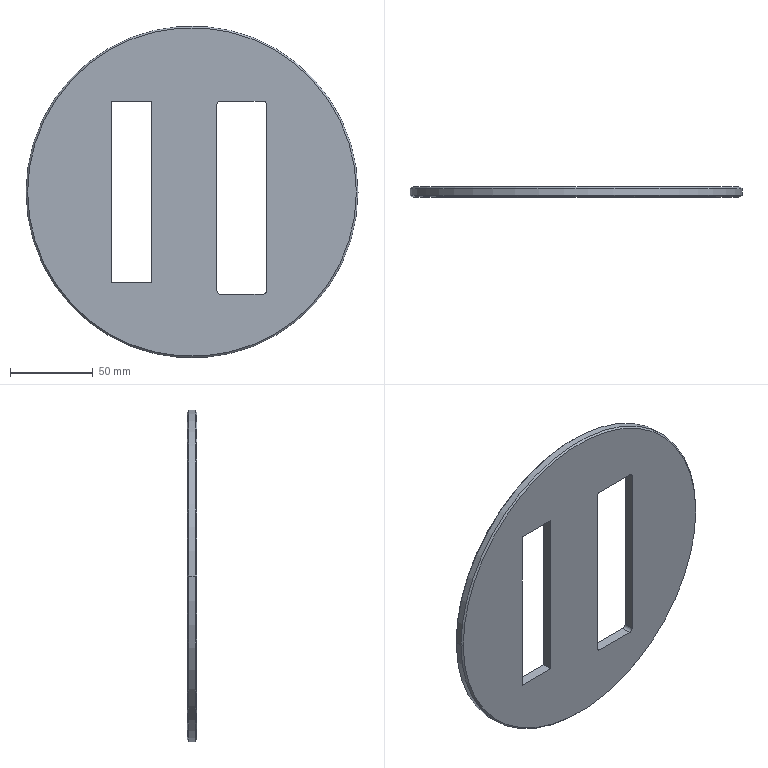Component | SolidWorks | Inline-H010-H01160308-003K-1 | 1 solid | 20 faces | box 200 x 6 x 200 mm | volume 151116 mm3 | plane 10 | cylinder 6 | cone 4 | commonest cylinder face diameters 4 x4 200 x2
build123d program:
from build123d import *

# Parameters (mm, degrees)
SKETCH1_R           = 100
BOSS_EXTRUDE1_DEPTH = 3
CHAMFER1_SIZE       = 1
SKETCH2_W           = 24.288
SKETCH2_H           = 109.389
CUT_EXTRUDE1_DEPTH  = 10


with BuildPart() as part:
    # Sketch1 → Boss-Extrude1 (new, symmetric)
    with BuildSketch(Plane.XY):
        Circle(SKETCH1_R)
    extrude(amount=BOSS_EXTRUDE1_DEPTH, both=True)

    # Chamfer1
    chamfer1_edges = [part.edges().sort_by_distance(p)[0] for p in [
        (-100, 0, -3),
        (-100, 0, 3),
    ]]
    chamfer(chamfer1_edges, length=CHAMFER1_SIZE)

    # Sketch2 → Cut-Extrude1 (cut)
    with BuildSketch(Plane(origin=(0, 0, -3), x_dir=(-1, 0, 0), z_dir=(0, 0, -1))):
        with BuildLine():
            Line((-17.028, -61.574), (-42.891, -61.574))
            ThreePointArc((-42.891, -61.574), (-44.305, -60.989), (-44.891, -59.574))
            Line((-44.891, -59.574), (-44.891, 52.695))
            ThreePointArc((-44.891, 52.695), (-44.305, 54.109), (-42.891, 54.695))
            Line((-42.891, 54.695), (-17.028, 54.695))
            ThreePointArc((-17.028, 54.695), (-15.614, 54.109), (-15.028, 52.695))
            Line((-15.028, 52.695), (-15.028, -59.574))
            ThreePointArc((-15.028, -59.574), (-15.614, -60.989), (-17.028, -61.574))
        make_face()
        with Locations((36.583, 0)):
            Rectangle(SKETCH2_W, SKETCH2_H)
    extrude(amount=-CUT_EXTRUDE1_DEPTH, mode=Mode.SUBTRACT)


solid = part.part

# Placed as in the assembly
solid = solid.moved(Location((29.082, 23.968, 139.665), (90, 0, 0)))
STEP:
#1=COLOUR_RGB('',0.7922,0.8196,0.9333);
#2=FILL_AREA_STYLE_COLOUR('',#1);
#3=FILL_AREA_STYLE('',(#2));
#4=SURFACE_STYLE_FILL_AREA(#3);
#5=SURFACE_SIDE_STYLE('',(#4));
#6=SURFACE_STYLE_USAGE(.BOTH.,#5);
#7=PRESENTATION_STYLE_ASSIGNMENT((#6));
#8=CARTESIAN_POINT('',(-2.753,1.062,5.499));
#9=VERTEX_POINT('',#8);
#10=CARTESIAN_POINT('',(5.043,1.062,5.499));
#11=VERTEX_POINT('',#10);
#12=CARTESIAN_POINT('',(1.145,1.062,5.499));
#13=DIRECTION('',(0.,1.,0.));
#14=DIRECTION('',(1.,-0.,0.));
#15=AXIS2_PLACEMENT_3D('',#12,#13,#14);
#16=CIRCLE('',#15,3.898);
#17=EDGE_CURVE('',#9,#11,#16,.T.);
#18=ORIENTED_EDGE('',*,*,#17,.F.);
#19=CARTESIAN_POINT('',(-2.792,1.022,5.499));
#20=VERTEX_POINT('',#19);
#21=CARTESIAN_POINT('',(-2.792,1.022,5.499));
#22=DIRECTION('',(-0.7071,-0.7071,0.));
#23=VECTOR('',#22,39.37);
#24=LINE('',#21,#23);
#25=EDGE_CURVE('',#9,#20,#24,.T.);
#26=ORIENTED_EDGE('',*,*,#25,.T.);
#27=CARTESIAN_POINT('',(5.082,1.022,5.499));
#28=VERTEX_POINT('',#27);
#29=CARTESIAN_POINT('',(1.145,1.022,5.499));
#30=DIRECTION('',(-0.,-1.,-0.));
#31=DIRECTION('',(1.,-0.,0.));
#32=AXIS2_PLACEMENT_3D('',#29,#30,#31);
#33=CIRCLE('',#32,3.937);
#34=EDGE_CURVE('',#28,#20,#33,.T.);
#35=ORIENTED_EDGE('',*,*,#34,.F.);
#36=CARTESIAN_POINT('',(5.082,1.022,5.499));
#37=DIRECTION('',(0.7071,-0.7071,-0.));
#38=VECTOR('',#37,39.37);
#39=LINE('',#36,#38);
#40=EDGE_CURVE('',#11,#28,#39,.T.);
#41=ORIENTED_EDGE('',*,*,#40,.F.);
#42=EDGE_LOOP('',(#18,#26,#35,#41));
#43=FACE_OUTER_BOUND('',#42,.T.);
#44=CARTESIAN_POINT('',(1.145,1.022,5.499));
#45=DIRECTION('',(-0.,-1.,-0.));
#46=DIRECTION('',(1.,-0.,0.));
#47=AXIS2_PLACEMENT_3D('',#44,#45,#46);
#48=CONICAL_SURFACE('',#47,3.937,0.7854);
#49=ADVANCED_FACE('',(#43),#48,.T.);
#50=CARTESIAN_POINT('',(5.043,0.8255,5.499));
#51=VERTEX_POINT('',#50);
#52=CARTESIAN_POINT('',(-2.753,0.8255,5.499));
#53=VERTEX_POINT('',#52);
#54=CARTESIAN_POINT('',(1.145,0.8255,5.499));
#55=DIRECTION('',(-0.,-1.,-0.));
#56=DIRECTION('',(1.,-0.,0.));
#57=AXIS2_PLACEMENT_3D('',#54,#55,#56);
#58=CIRCLE('',#57,3.898);
#59=EDGE_CURVE('',#51,#53,#58,.T.);
#60=ORIENTED_EDGE('',*,*,#59,.F.);
#61=CARTESIAN_POINT('',(5.082,0.8649,5.499));
#62=VERTEX_POINT('',#61);
#63=CARTESIAN_POINT('',(5.043,0.8255,5.499));
#64=DIRECTION('',(0.7071,0.7071,0.));
#65=VECTOR('',#64,39.37);
#66=LINE('',#63,#65);
#67=EDGE_CURVE('',#51,#62,#66,.T.);
#68=ORIENTED_EDGE('',*,*,#67,.T.);
#69=CARTESIAN_POINT('',(-2.792,0.8649,5.499));
#70=VERTEX_POINT('',#69);
#71=CARTESIAN_POINT('',(1.145,0.8649,5.499));
#72=DIRECTION('',(0.,1.,0.));
#73=DIRECTION('',(1.,-0.,0.));
#74=AXIS2_PLACEMENT_3D('',#71,#72,#73);
#75=CIRCLE('',#74,3.937);
#76=EDGE_CURVE('',#70,#62,#75,.T.);
#77=ORIENTED_EDGE('',*,*,#76,.F.);
#78=CARTESIAN_POINT('',(-2.753,0.8255,5.499));
#79=DIRECTION('',(-0.7071,0.7071,0.));
#80=VECTOR('',#79,39.37);
#81=LINE('',#78,#80);
#82=EDGE_CURVE('',#53,#70,#81,.T.);
#83=ORIENTED_EDGE('',*,*,#82,.F.);
#84=EDGE_LOOP('',(#60,#68,#77,#83));
#85=FACE_OUTER_BOUND('',#84,.T.);
#86=CARTESIAN_POINT('',(1.145,0.8255,5.499));
#87=DIRECTION('',(0.,1.,0.));
#88=DIRECTION('',(-1.,0.,0.));
#89=AXIS2_PLACEMENT_3D('',#86,#87,#88);
#90=CONICAL_SURFACE('',#89,3.898,0.7854);
#91=ADVANCED_FACE('',(#85),#90,.T.);
#92=ORIENTED_EDGE('',*,*,#76,.T.);
#93=CARTESIAN_POINT('',(5.082,0.8255,5.499));
#94=DIRECTION('',(0.,1.,0.));
#95=VECTOR('',#94,39.37);
#96=LINE('',#93,#95);
#97=EDGE_CURVE('',#62,#28,#96,.T.);
#98=ORIENTED_EDGE('',*,*,#97,.T.);
#99=ORIENTED_EDGE('',*,*,#34,.T.);
#100=CARTESIAN_POINT('',(-2.792,0.8255,5.499));
#101=DIRECTION('',(0.,1.,0.));
#102=VECTOR('',#101,39.37);
#103=LINE('',#100,#102);
#104=EDGE_CURVE('',#70,#20,#103,.T.);
#105=ORIENTED_EDGE('',*,*,#104,.F.);
#106=EDGE_LOOP('',(#92,#98,#99,#105));
#107=FACE_OUTER_BOUND('',#106,.T.);
#108=CARTESIAN_POINT('',(1.145,0.8255,5.499));
#109=DIRECTION('',(0.,1.,0.));
#110=DIRECTION('',(-1.,0.,0.));
#111=AXIS2_PLACEMENT_3D('',#108,#109,#110);
#112=CYLINDRICAL_SURFACE('',#111,3.937);
#113=ADVANCED_FACE('',(#107),#112,.T.);
#114=ORIENTED_EDGE('',*,*,#97,.F.);
#115=CARTESIAN_POINT('',(1.145,0.8649,5.499));
#116=DIRECTION('',(0.,1.,0.));
#117=DIRECTION('',(1.,-0.,0.));
#118=AXIS2_PLACEMENT_3D('',#115,#116,#117);
#119=CIRCLE('',#118,3.937);
#120=EDGE_CURVE('',#62,#70,#119,.T.);
#121=ORIENTED_EDGE('',*,*,#120,.T.);
#122=ORIENTED_EDGE('',*,*,#104,.T.);
#123=CARTESIAN_POINT('',(1.145,1.022,5.499));
#124=DIRECTION('',(-0.,-1.,-0.));
#125=DIRECTION('',(1.,-0.,0.));
#126=AXIS2_PLACEMENT_3D('',#123,#124,#125);
#127=CIRCLE('',#126,3.937);
#128=EDGE_CURVE('',#20,#28,#127,.T.);
#129=ORIENTED_EDGE('',*,*,#128,.T.);
#130=EDGE_LOOP('',(#114,#121,#122,#129));
#131=FACE_OUTER_BOUND('',#130,.T.);
#132=CARTESIAN_POINT('',(1.145,0.8255,5.499));
#133=DIRECTION('',(0.,1.,0.));
#134=DIRECTION('',(-1.,0.,0.));
#135=AXIS2_PLACEMENT_3D('',#132,#133,#134);
#136=CYLINDRICAL_SURFACE('',#135,3.937);
#137=ADVANCED_FACE('',(#131),#136,.T.);
#138=CARTESIAN_POINT('',(0.1828,0.8255,3.345));
#139=VERTEX_POINT('',#138);
#140=CARTESIAN_POINT('',(0.1828,0.8255,7.652));
#141=VERTEX_POINT('',#140);
#142=CARTESIAN_POINT('',(0.1828,0.8255,5.499));
#143=DIRECTION('',(0.,-0.,1.));
#144=VECTOR('',#143,39.37);
#145=LINE('',#142,#144);
#146=EDGE_CURVE('',#139,#141,#145,.T.);
#147=ORIENTED_EDGE('',*,*,#146,.F.);
#148=CARTESIAN_POINT('',(-0.7734,0.8255,3.345));
#149=VERTEX_POINT('',#148);
#150=CARTESIAN_POINT('',(1.145,0.8255,3.345));
#151=DIRECTION('',(1.,-0.,-0.));
#152=VECTOR('',#151,39.37);
#153=LINE('',#150,#152);
#154=EDGE_CURVE('',#149,#139,#153,.T.);
#155=ORIENTED_EDGE('',*,*,#154,.F.);
#156=CARTESIAN_POINT('',(-0.7734,0.8255,7.652));
#157=VERTEX_POINT('',#156);
#158=CARTESIAN_POINT('',(-0.7734,0.8255,5.499));
#159=DIRECTION('',(-0.,0.,-1.));
#160=VECTOR('',#159,39.37);
#161=LINE('',#158,#160);
#162=EDGE_CURVE('',#157,#149,#161,.T.);
#163=ORIENTED_EDGE('',*,*,#162,.F.);
#164=CARTESIAN_POINT('',(1.145,0.8255,7.652));
#165=DIRECTION('',(-1.,0.,0.));
#166=VECTOR('',#165,39.37);
#167=LINE('',#164,#166);
#168=EDGE_CURVE('',#141,#157,#167,.T.);
#169=ORIENTED_EDGE('',*,*,#168,.F.);
#170=EDGE_LOOP('',(#147,#155,#163,#169));
#171=FACE_BOUND('',#170,.T.);
#172=CARTESIAN_POINT('',(1.737,0.8255,3.153));
#173=VERTEX_POINT('',#172);
#174=CARTESIAN_POINT('',(1.815,0.8255,3.074));
#175=VERTEX_POINT('',#174);
#176=CARTESIAN_POINT('',(1.815,0.8255,3.153));
#177=DIRECTION('',(-0.,-1.,-0.));
#178=DIRECTION('',(1.,0.,0.));
#179=AXIS2_PLACEMENT_3D('',#176,#177,#178);
#180=CIRCLE('',#179,0.07874);
#181=EDGE_CURVE('',#173,#175,#180,.T.);
#182=ORIENTED_EDGE('',*,*,#181,.F.);
#183=CARTESIAN_POINT('',(1.737,0.8255,7.573));
#184=VERTEX_POINT('',#183);
#185=CARTESIAN_POINT('',(1.737,0.8255,5.499));
#186=DIRECTION('',(-0.,0.,-1.));
#187=VECTOR('',#186,39.37);
#188=LINE('',#185,#187);
#189=EDGE_CURVE('',#184,#173,#188,.T.);
#190=ORIENTED_EDGE('',*,*,#189,.F.);
#191=CARTESIAN_POINT('',(1.815,0.8255,7.652));
#192=VERTEX_POINT('',#191);
#193=CARTESIAN_POINT('',(1.815,0.8255,7.573));
#194=DIRECTION('',(-0.,-1.,-0.));
#195=DIRECTION('',(1.,0.,0.));
#196=AXIS2_PLACEMENT_3D('',#193,#194,#195);
#197=CIRCLE('',#196,0.07874);
#198=EDGE_CURVE('',#192,#184,#197,.T.);
#199=ORIENTED_EDGE('',*,*,#198,.F.);
#200=CARTESIAN_POINT('',(2.834,0.8255,7.652));
#201=VERTEX_POINT('',#200);
#202=CARTESIAN_POINT('',(1.145,0.8255,7.652));
#203=DIRECTION('',(-1.,0.,0.));
#204=VECTOR('',#203,39.37);
#205=LINE('',#202,#204);
#206=EDGE_CURVE('',#201,#192,#205,.T.);
#207=ORIENTED_EDGE('',*,*,#206,.F.);
#208=CARTESIAN_POINT('',(2.912,0.8255,7.573));
#209=VERTEX_POINT('',#208);
#210=CARTESIAN_POINT('',(2.834,0.8255,7.573));
#211=DIRECTION('',(-0.,-1.,-0.));
#212=DIRECTION('',(1.,0.,0.));
#213=AXIS2_PLACEMENT_3D('',#210,#211,#212);
#214=CIRCLE('',#213,0.07874);
#215=EDGE_CURVE('',#209,#201,#214,.T.);
#216=ORIENTED_EDGE('',*,*,#215,.F.);
#217=CARTESIAN_POINT('',(2.912,0.8255,3.153));
#218=VERTEX_POINT('',#217);
#219=CARTESIAN_POINT('',(2.912,0.8255,5.499));
#220=DIRECTION('',(0.,-0.,1.));
#221=VECTOR('',#220,39.37);
#222=LINE('',#219,#221);
#223=EDGE_CURVE('',#218,#209,#222,.T.);
#224=ORIENTED_EDGE('',*,*,#223,.F.);
#225=CARTESIAN_POINT('',(2.834,0.8255,3.074));
#226=VERTEX_POINT('',#225);
#227=CARTESIAN_POINT('',(2.834,0.8255,3.153));
#228=DIRECTION('',(-0.,-1.,-0.));
#229=DIRECTION('',(1.,0.,0.));
#230=AXIS2_PLACEMENT_3D('',#227,#228,#229);
#231=CIRCLE('',#230,0.07874);
#232=EDGE_CURVE('',#226,#218,#231,.T.);
#233=ORIENTED_EDGE('',*,*,#232,.F.);
#234=CARTESIAN_POINT('',(1.145,0.8255,3.074));
#235=DIRECTION('',(1.,-0.,-0.));
#236=VECTOR('',#235,39.37);
#237=LINE('',#234,#236);
#238=EDGE_CURVE('',#175,#226,#237,.T.);
#239=ORIENTED_EDGE('',*,*,#238,.F.);
#240=EDGE_LOOP('',(#182,#190,#199,#207,#216,#224,#233,#239));
#241=FACE_BOUND('',#240,.T.);
#242=CARTESIAN_POINT('',(1.145,0.8255,5.499));
#243=DIRECTION('',(-0.,-1.,-0.));
#244=DIRECTION('',(1.,-0.,0.));
#245=AXIS2_PLACEMENT_3D('',#242,#243,#244);
#246=CIRCLE('',#245,3.898);
#247=EDGE_CURVE('',#53,#51,#246,.T.);
#248=ORIENTED_EDGE('',*,*,#247,.T.);
#249=ORIENTED_EDGE('',*,*,#59,.T.);
#250=EDGE_LOOP('',(#248,#249));
#251=FACE_OUTER_BOUND('',#250,.T.);
#252=CARTESIAN_POINT('',(1.145,0.8255,5.499));
#253=DIRECTION('',(-0.,-1.,-0.));
#254=DIRECTION('',(1.,-0.,-0.));
#255=AXIS2_PLACEMENT_3D('',#252,#253,#254);
#256=PLANE('',#255);
#257=ADVANCED_FACE('',(#171,#241,#251),#256,.T.);
#258=CARTESIAN_POINT('',(0.1828,1.062,3.345));
#259=VERTEX_POINT('',#258);
#260=CARTESIAN_POINT('',(-0.7734,1.062,3.345));
#261=VERTEX_POINT('',#260);
#262=CARTESIAN_POINT('',(-0.7734,1.062,3.345));
#263=DIRECTION('',(-1.,0.,0.));
#264=VECTOR('',#263,39.37);
#265=LINE('',#262,#264);
#266=EDGE_CURVE('',#259,#261,#265,.T.);
#267=ORIENTED_EDGE('',*,*,#266,.F.);
#268=CARTESIAN_POINT('',(0.1828,1.062,7.652));
#269=VERTEX_POINT('',#268);
#270=CARTESIAN_POINT('',(0.1828,1.062,3.345));
#271=DIRECTION('',(-0.,0.,-1.));
#272=VECTOR('',#271,39.37);
#273=LINE('',#270,#272);
#274=EDGE_CURVE('',#269,#259,#273,.T.);
#275=ORIENTED_EDGE('',*,*,#274,.F.);
#276=CARTESIAN_POINT('',(-0.7734,1.062,7.652));
#277=VERTEX_POINT('',#276);
#278=CARTESIAN_POINT('',(-0.7734,1.062,7.652));
#279=DIRECTION('',(1.,-0.,-0.));
#280=VECTOR('',#279,39.37);
#281=LINE('',#278,#280);
#282=EDGE_CURVE('',#277,#269,#281,.T.);
#283=ORIENTED_EDGE('',*,*,#282,.F.);
#284=CARTESIAN_POINT('',(-0.7734,1.062,3.345));
#285=DIRECTION('',(0.,-0.,1.));
#286=VECTOR('',#285,39.37);
#287=LINE('',#284,#286);
#288=EDGE_CURVE('',#261,#277,#287,.T.);
#289=ORIENTED_EDGE('',*,*,#288,.F.);
#290=EDGE_LOOP('',(#267,#275,#283,#289));
#291=FACE_BOUND('',#290,.T.);
#292=CARTESIAN_POINT('',(1.737,1.062,3.153));
#293=VERTEX_POINT('',#292);
#294=CARTESIAN_POINT('',(1.737,1.062,7.573));
#295=VERTEX_POINT('',#294);
#296=CARTESIAN_POINT('',(1.737,1.062,3.153));
#297=DIRECTION('',(0.,-0.,1.));
#298=VECTOR('',#297,39.37);
#299=LINE('',#296,#298);
#300=EDGE_CURVE('',#293,#295,#299,.T.);
#301=ORIENTED_EDGE('',*,*,#300,.F.);
#302=CARTESIAN_POINT('',(1.815,1.062,3.074));
#303=VERTEX_POINT('',#302);
#304=CARTESIAN_POINT('',(1.815,1.062,3.153));
#305=DIRECTION('',(0.,1.,0.));
#306=DIRECTION('',(-1.,0.,0.));
#307=AXIS2_PLACEMENT_3D('',#304,#305,#306);
#308=CIRCLE('',#307,0.07874);
#309=EDGE_CURVE('',#303,#293,#308,.T.);
#310=ORIENTED_EDGE('',*,*,#309,.F.);
#311=CARTESIAN_POINT('',(2.834,1.062,3.074));
#312=VERTEX_POINT('',#311);
#313=CARTESIAN_POINT('',(1.815,1.062,3.074));
#314=DIRECTION('',(-1.,0.,0.));
#315=VECTOR('',#314,39.37);
#316=LINE('',#313,#315);
#317=EDGE_CURVE('',#312,#303,#316,.T.);
#318=ORIENTED_EDGE('',*,*,#317,.F.);
#319=CARTESIAN_POINT('',(2.912,1.062,3.153));
#320=VERTEX_POINT('',#319);
#321=CARTESIAN_POINT('',(2.834,1.062,3.153));
#322=DIRECTION('',(0.,1.,0.));
#323=DIRECTION('',(1.,0.,0.));
#324=AXIS2_PLACEMENT_3D('',#321,#322,#323);
#325=CIRCLE('',#324,0.07874);
#326=EDGE_CURVE('',#320,#312,#325,.T.);
#327=ORIENTED_EDGE('',*,*,#326,.F.);
#328=CARTESIAN_POINT('',(2.912,1.062,7.573));
#329=VERTEX_POINT('',#328);
#330=CARTESIAN_POINT('',(2.912,1.062,3.153));
#331=DIRECTION('',(-0.,0.,-1.));
#332=VECTOR('',#331,39.37);
#333=LINE('',#330,#332);
#334=EDGE_CURVE('',#329,#320,#333,.T.);
#335=ORIENTED_EDGE('',*,*,#334,.F.);
#336=CARTESIAN_POINT('',(2.834,1.062,7.652));
#337=VERTEX_POINT('',#336);
#338=CARTESIAN_POINT('',(2.834,1.062,7.573));
#339=DIRECTION('',(0.,1.,0.));
#340=DIRECTION('',(-1.,0.,0.));
#341=AXIS2_PLACEMENT_3D('',#338,#339,#340);
#342=CIRCLE('',#341,0.07874);
#343=EDGE_CURVE('',#337,#329,#342,.T.);
#344=ORIENTED_EDGE('',*,*,#343,.F.);
#345=CARTESIAN_POINT('',(1.815,1.062,7.652));
#346=VERTEX_POINT('',#345);
#347=CARTESIAN_POINT('',(1.815,1.062,7.652));
#348=DIRECTION('',(1.,-0.,-0.));
#349=VECTOR('',#348,39.37);
#350=LINE('',#347,#349);
#351=EDGE_CURVE('',#346,#337,#350,.T.);
#352=ORIENTED_EDGE('',*,*,#351,.F.);
#353=CARTESIAN_POINT('',(1.815,1.062,7.573));
#354=DIRECTION('',(0.,1.,0.));
#355=DIRECTION('',(-1.,0.,0.));
#356=AXIS2_PLACEMENT_3D('',#353,#354,#355);
#357=CIRCLE('',#356,0.07874);
#358=EDGE_CURVE('',#295,#346,#357,.T.);
#359=ORIENTED_EDGE('',*,*,#358,.F.);
#360=EDGE_LOOP('',(#301,#310,#318,#327,#335,#344,#352,#359));
#361=FACE_BOUND('',#360,.T.);
#362=CARTESIAN_POINT('',(1.145,1.062,5.499));
#363=DIRECTION('',(0.,1.,0.));
#364=DIRECTION('',(1.,-0.,0.));
#365=AXIS2_PLACEMENT_3D('',#362,#363,#364);
#366=CIRCLE('',#365,3.898);
#367=EDGE_CURVE('',#11,#9,#366,.T.);
#368=ORIENTED_EDGE('',*,*,#367,.T.);
#369=ORIENTED_EDGE('',*,*,#17,.T.);
#370=EDGE_LOOP('',(#368,#369));
#371=FACE_OUTER_BOUND('',#370,.T.);
#372=CARTESIAN_POINT('',(1.145,1.062,5.499));
#373=DIRECTION('',(-0.,-1.,-0.));
#374=DIRECTION('',(1.,-0.,-0.));
#375=AXIS2_PLACEMENT_3D('',#372,#373,#374);
#376=PLANE('',#375);
#377=ADVANCED_FACE('',(#291,#361,#371),#376,.F.);
#378=ORIENTED_EDGE('',*,*,#67,.F.);
#379=ORIENTED_EDGE('',*,*,#247,.F.);
#380=ORIENTED_EDGE('',*,*,#82,.T.);
#381=ORIENTED_EDGE('',*,*,#120,.F.);
#382=EDGE_LOOP('',(#378,#379,#380,#381));
#383=FACE_OUTER_BOUND('',#382,.T.);
#384=CARTESIAN_POINT('',(1.145,0.8255,5.499));
#385=DIRECTION('',(0.,1.,0.));
#386=DIRECTION('',(-1.,0.,0.));
#387=AXIS2_PLACEMENT_3D('',#384,#385,#386);
#388=CONICAL_SURFACE('',#387,3.898,0.7854);
#389=ADVANCED_FACE('',(#383),#388,.T.);
#390=ORIENTED_EDGE('',*,*,#25,.F.);
#391=ORIENTED_EDGE('',*,*,#367,.F.);
#392=ORIENTED_EDGE('',*,*,#40,.T.);
#393=ORIENTED_EDGE('',*,*,#128,.F.);
#394=EDGE_LOOP('',(#390,#391,#392,#393));
#395=FACE_OUTER_BOUND('',#394,.T.);
#396=CARTESIAN_POINT('',(1.145,1.022,5.499));
#397=DIRECTION('',(-0.,-1.,-0.));
#398=DIRECTION('',(1.,-0.,0.));
#399=AXIS2_PLACEMENT_3D('',#396,#397,#398);
#400=CONICAL_SURFACE('',#399,3.937,0.7854);
#401=ADVANCED_FACE('',(#395),#400,.T.);
#402=ORIENTED_EDGE('',*,*,#181,.T.);
#403=CARTESIAN_POINT('',(1.815,0.668,3.074));
#404=DIRECTION('',(0.,1.,0.));
#405=VECTOR('',#404,39.37);
#406=LINE('',#403,#405);
#407=EDGE_CURVE('',#175,#303,#406,.T.);
#408=ORIENTED_EDGE('',*,*,#407,.T.);
#409=ORIENTED_EDGE('',*,*,#309,.T.);
#410=CARTESIAN_POINT('',(1.737,0.668,3.153));
#411=DIRECTION('',(0.,1.,0.));
#412=VECTOR('',#411,39.37);
#413=LINE('',#410,#412);
#414=EDGE_CURVE('',#173,#293,#413,.T.);
#415=ORIENTED_EDGE('',*,*,#414,.F.);
#416=EDGE_LOOP('',(#402,#408,#409,#415));
#417=FACE_OUTER_BOUND('',#416,.T.);
#418=CARTESIAN_POINT('',(1.815,0.668,3.153));
#419=DIRECTION('',(0.,1.,0.));
#420=DIRECTION('',(-1.,0.,0.));
#421=AXIS2_PLACEMENT_3D('',#418,#419,#420);
#422=CYLINDRICAL_SURFACE('',#421,0.07874);
#423=ADVANCED_FACE('',(#417),#422,.F.);
#424=ORIENTED_EDGE('',*,*,#238,.T.);
#425=CARTESIAN_POINT('',(2.834,0.668,3.074));
#426=DIRECTION('',(0.,1.,0.));
#427=VECTOR('',#426,39.37);
#428=LINE('',#425,#427);
#429=EDGE_CURVE('',#226,#312,#428,.T.);
#430=ORIENTED_EDGE('',*,*,#429,.T.);
#431=ORIENTED_EDGE('',*,*,#317,.T.);
#432=ORIENTED_EDGE('',*,*,#407,.F.);
#433=EDGE_LOOP('',(#424,#430,#431,#432));
#434=FACE_OUTER_BOUND('',#433,.T.);
#435=CARTESIAN_POINT('',(1.815,0.668,3.074));
#436=DIRECTION('',(-0.,0.,-1.));
#437=DIRECTION('',(0.,1.,0.));
#438=AXIS2_PLACEMENT_3D('',#435,#436,#437);
#439=PLANE('',#438);
#440=ADVANCED_FACE('',(#434),#439,.F.);
#441=ORIENTED_EDGE('',*,*,#232,.T.);
#442=CARTESIAN_POINT('',(2.912,0.668,3.153));
#443=DIRECTION('',(0.,1.,0.));
#444=VECTOR('',#443,39.37);
#445=LINE('',#442,#444);
#446=EDGE_CURVE('',#218,#320,#445,.T.);
#447=ORIENTED_EDGE('',*,*,#446,.T.);
#448=ORIENTED_EDGE('',*,*,#326,.T.);
#449=ORIENTED_EDGE('',*,*,#429,.F.);
#450=EDGE_LOOP('',(#441,#447,#448,#449));
#451=FACE_OUTER_BOUND('',#450,.T.);
#452=CARTESIAN_POINT('',(2.834,0.668,3.153));
#453=DIRECTION('',(0.,1.,0.));
#454=DIRECTION('',(-1.,0.,0.));
#455=AXIS2_PLACEMENT_3D('',#452,#453,#454);
#456=CYLINDRICAL_SURFACE('',#455,0.07874);
#457=ADVANCED_FACE('',(#451),#456,.F.);
#458=ORIENTED_EDGE('',*,*,#223,.T.);
#459=CARTESIAN_POINT('',(2.912,0.668,7.573));
#460=DIRECTION('',(0.,1.,0.));
#461=VECTOR('',#460,39.37);
#462=LINE('',#459,#461);
#463=EDGE_CURVE('',#209,#329,#462,.T.);
#464=ORIENTED_EDGE('',*,*,#463,.T.);
#465=ORIENTED_EDGE('',*,*,#334,.T.);
#466=ORIENTED_EDGE('',*,*,#446,.F.);
#467=EDGE_LOOP('',(#458,#464,#465,#466));
#468=FACE_OUTER_BOUND('',#467,.T.);
#469=CARTESIAN_POINT('',(2.912,0.668,3.153));
#470=DIRECTION('',(1.,-0.,-0.));
#471=DIRECTION('',(0.,1.,0.));
#472=AXIS2_PLACEMENT_3D('',#469,#470,#471);
#473=PLANE('',#472);
#474=ADVANCED_FACE('',(#468),#473,.F.);
#475=ORIENTED_EDGE('',*,*,#215,.T.);
#476=CARTESIAN_POINT('',(2.834,0.668,7.652));
#477=DIRECTION('',(0.,1.,0.));
#478=VECTOR('',#477,39.37);
#479=LINE('',#476,#478);
#480=EDGE_CURVE('',#201,#337,#479,.T.);
#481=ORIENTED_EDGE('',*,*,#480,.T.);
#482=ORIENTED_EDGE('',*,*,#343,.T.);
#483=ORIENTED_EDGE('',*,*,#463,.F.);
#484=EDGE_LOOP('',(#475,#481,#482,#483));
#485=FACE_OUTER_BOUND('',#484,.T.);
#486=CARTESIAN_POINT('',(2.834,0.668,7.573));
#487=DIRECTION('',(0.,1.,0.));
#488=DIRECTION('',(-1.,0.,0.));
#489=AXIS2_PLACEMENT_3D('',#486,#487,#488);
#490=CYLINDRICAL_SURFACE('',#489,0.07874);
#491=ADVANCED_FACE('',(#485),#490,.F.);
#492=ORIENTED_EDGE('',*,*,#206,.T.);
#493=CARTESIAN_POINT('',(1.815,0.668,7.652));
#494=DIRECTION('',(0.,1.,0.));
#495=VECTOR('',#494,39.37);
#496=LINE('',#493,#495);
#497=EDGE_CURVE('',#192,#346,#496,.T.);
#498=ORIENTED_EDGE('',*,*,#497,.T.);
#499=ORIENTED_EDGE('',*,*,#351,.T.);
#500=ORIENTED_EDGE('',*,*,#480,.F.);
#501=EDGE_LOOP('',(#492,#498,#499,#500));
#502=FACE_OUTER_BOUND('',#501,.T.);
#503=CARTESIAN_POINT('',(1.815,0.668,7.652));
#504=DIRECTION('',(0.,-0.,1.));
#505=DIRECTION('',(-0.,-1.,-0.));
#506=AXIS2_PLACEMENT_3D('',#503,#504,#505);
#507=PLANE('',#506);
#508=ADVANCED_FACE('',(#502),#507,.F.);
#509=ORIENTED_EDGE('',*,*,#198,.T.);
#510=CARTESIAN_POINT('',(1.737,0.668,7.573));
#511=DIRECTION('',(0.,1.,0.));
#512=VECTOR('',#511,39.37);
#513=LINE('',#510,#512);
#514=EDGE_CURVE('',#184,#295,#513,.T.);
#515=ORIENTED_EDGE('',*,*,#514,.T.);
#516=ORIENTED_EDGE('',*,*,#358,.T.);
#517=ORIENTED_EDGE('',*,*,#497,.F.);
#518=EDGE_LOOP('',(#509,#515,#516,#517));
#519=FACE_OUTER_BOUND('',#518,.T.);
#520=CARTESIAN_POINT('',(1.815,0.668,7.573));
#521=DIRECTION('',(0.,1.,0.));
#522=DIRECTION('',(-1.,0.,0.));
#523=AXIS2_PLACEMENT_3D('',#520,#521,#522);
#524=CYLINDRICAL_SURFACE('',#523,0.07874);
#525=ADVANCED_FACE('',(#519),#524,.F.);
#526=ORIENTED_EDGE('',*,*,#189,.T.);
#527=ORIENTED_EDGE('',*,*,#414,.T.);
#528=ORIENTED_EDGE('',*,*,#300,.T.);
#529=ORIENTED_EDGE('',*,*,#514,.F.);
#530=EDGE_LOOP('',(#526,#527,#528,#529));
#531=FACE_OUTER_BOUND('',#530,.T.);
#532=CARTESIAN_POINT('',(1.737,0.668,3.153));
#533=DIRECTION('',(-1.,0.,0.));
#534=DIRECTION('',(-0.,-1.,-0.));
#535=AXIS2_PLACEMENT_3D('',#532,#533,#534);
#536=PLANE('',#535);
#537=ADVANCED_FACE('',(#531),#536,.F.);
#538=ORIENTED_EDGE('',*,*,#146,.T.);
#539=CARTESIAN_POINT('',(0.1828,0.668,7.652));
#540=DIRECTION('',(0.,1.,0.));
#541=VECTOR('',#540,39.37);
#542=LINE('',#539,#541);
#543=EDGE_CURVE('',#141,#269,#542,.T.);
#544=ORIENTED_EDGE('',*,*,#543,.T.);
#545=ORIENTED_EDGE('',*,*,#274,.T.);
#546=CARTESIAN_POINT('',(0.1828,0.668,3.345));
#547=DIRECTION('',(0.,1.,0.));
#548=VECTOR('',#547,39.37);
#549=LINE('',#546,#548);
#550=EDGE_CURVE('',#139,#259,#549,.T.);
#551=ORIENTED_EDGE('',*,*,#550,.F.);
#552=EDGE_LOOP('',(#538,#544,#545,#551));
#553=FACE_OUTER_BOUND('',#552,.T.);
#554=CARTESIAN_POINT('',(0.1828,0.668,3.345));
#555=DIRECTION('',(1.,-0.,-0.));
#556=DIRECTION('',(0.,1.,0.));
#557=AXIS2_PLACEMENT_3D('',#554,#555,#556);
#558=PLANE('',#557);
#559=ADVANCED_FACE('',(#553),#558,.F.);
#560=ORIENTED_EDGE('',*,*,#168,.T.);
#561=CARTESIAN_POINT('',(-0.7734,0.668,7.652));
#562=DIRECTION('',(0.,1.,0.));
#563=VECTOR('',#562,39.37);
#564=LINE('',#561,#563);
#565=EDGE_CURVE('',#157,#277,#564,.T.);
#566=ORIENTED_EDGE('',*,*,#565,.T.);
#567=ORIENTED_EDGE('',*,*,#282,.T.);
#568=ORIENTED_EDGE('',*,*,#543,.F.);
#569=EDGE_LOOP('',(#560,#566,#567,#568));
#570=FACE_OUTER_BOUND('',#569,.T.);
#571=CARTESIAN_POINT('',(-0.7734,0.668,7.652));
#572=DIRECTION('',(0.,-0.,1.));
#573=DIRECTION('',(-0.,-1.,-0.));
#574=AXIS2_PLACEMENT_3D('',#571,#572,#573);
#575=PLANE('',#574);
#576=ADVANCED_FACE('',(#570),#575,.F.);
#577=ORIENTED_EDGE('',*,*,#162,.T.);
#578=CARTESIAN_POINT('',(-0.7734,0.668,3.345));
#579=DIRECTION('',(0.,1.,0.));
#580=VECTOR('',#579,39.37);
#581=LINE('',#578,#580);
#582=EDGE_CURVE('',#149,#261,#581,.T.);
#583=ORIENTED_EDGE('',*,*,#582,.T.);
#584=ORIENTED_EDGE('',*,*,#288,.T.);
#585=ORIENTED_EDGE('',*,*,#565,.F.);
#586=EDGE_LOOP('',(#577,#583,#584,#585));
#587=FACE_OUTER_BOUND('',#586,.T.);
#588=CARTESIAN_POINT('',(-0.7734,0.668,3.345));
#589=DIRECTION('',(-1.,0.,0.));
#590=DIRECTION('',(-0.,-1.,-0.));
#591=AXIS2_PLACEMENT_3D('',#588,#589,#590);
#592=PLANE('',#591);
#593=ADVANCED_FACE('',(#587),#592,.F.);
#594=ORIENTED_EDGE('',*,*,#154,.T.);
#595=ORIENTED_EDGE('',*,*,#550,.T.);
#596=ORIENTED_EDGE('',*,*,#266,.T.);
#597=ORIENTED_EDGE('',*,*,#582,.F.);
#598=EDGE_LOOP('',(#594,#595,#596,#597));
#599=FACE_OUTER_BOUND('',#598,.T.);
#600=CARTESIAN_POINT('',(-0.7734,0.668,3.345));
#601=DIRECTION('',(-0.,0.,-1.));
#602=DIRECTION('',(0.,1.,0.));
#603=AXIS2_PLACEMENT_3D('',#600,#601,#602);
#604=PLANE('',#603);
#605=ADVANCED_FACE('',(#599),#604,.F.);
#606=CLOSED_SHELL('',(#49,#91,#113,#137,#257,#377,#389,#401,#423,#440,#457,#474,#491,#508,#525,#537,#559,#576,#593,#605));
#607=MANIFOLD_SOLID_BREP('',#606);
#608=STYLED_ITEM('',(#7),#607);
#609=PRESENTATION_LAYER_ASSIGNMENT('','',(#608));
#610=CARTESIAN_POINT('',(0.,0.,0.));
#611=DIRECTION('',(0.,0.,1.));
#612=DIRECTION('',(1.,0.,0.));
#613=AXIS2_PLACEMENT_3D('',#610,#611,#612);
#614=(LENGTH_UNIT()NAMED_UNIT(*)SI_UNIT($,.METRE.));
#615=LENGTH_MEASURE_WITH_UNIT(LENGTH_MEASURE(0.0254),#614);
#616=DIMENSIONAL_EXPONENTS(1.,0.,0.,0.,0.,0.,0.);
#617=(CONVERSION_BASED_UNIT('',#615)LENGTH_UNIT()NAMED_UNIT(#616));
#618=UNCERTAINTY_MEASURE_WITH_UNIT(LENGTH_MEASURE(0.00001),#617,'','');
#619=(NAMED_UNIT(*)PLANE_ANGLE_UNIT()SI_UNIT($,.RADIAN.));
#620=(NAMED_UNIT(*)SI_UNIT($,.STERADIAN.)SOLID_ANGLE_UNIT());
#621=(GEOMETRIC_REPRESENTATION_CONTEXT(3)GLOBAL_UNCERTAINTY_ASSIGNED_CONTEXT((#618))GLOBAL_UNIT_ASSIGNED_CONTEXT((#617,#619,#620))REPRESENTATION_CONTEXT('',''));
#622=ADVANCED_BREP_SHAPE_REPRESENTATION('',(#607,#613),#621);
#623=(LENGTH_UNIT()NAMED_UNIT(*)SI_UNIT($,.METRE.));
#624=LENGTH_MEASURE_WITH_UNIT(LENGTH_MEASURE(0.0254),#623);
#625=DIMENSIONAL_EXPONENTS(1.,0.,0.,0.,0.,0.,0.);
#626=(CONVERSION_BASED_UNIT('',#624)LENGTH_UNIT()NAMED_UNIT(#625));
#627=UNCERTAINTY_MEASURE_WITH_UNIT(LENGTH_MEASURE(0.00001),#626,'','');
#628=(NAMED_UNIT(*)PLANE_ANGLE_UNIT()SI_UNIT($,.RADIAN.));
#629=(NAMED_UNIT(*)SI_UNIT($,.STERADIAN.)SOLID_ANGLE_UNIT());
#630=(GEOMETRIC_REPRESENTATION_CONTEXT(3)GLOBAL_UNCERTAINTY_ASSIGNED_CONTEXT((#627))GLOBAL_UNIT_ASSIGNED_CONTEXT((#626,#628,#629))REPRESENTATION_CONTEXT('',''));
#631=MECHANICAL_DESIGN_GEOMETRIC_PRESENTATION_REPRESENTATION('',(#608),#630);